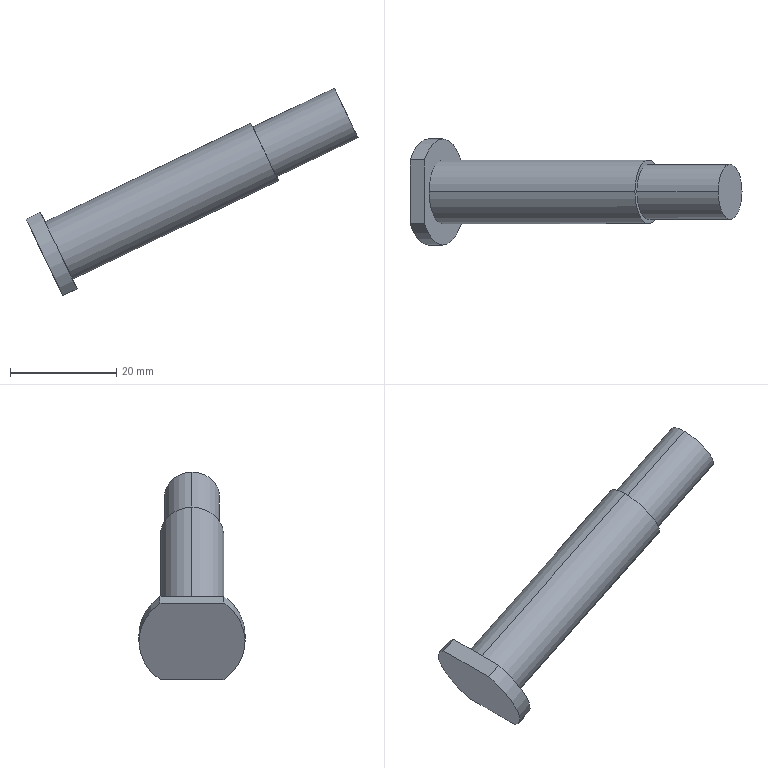Component | SolidWorks | DowelPin1-1-2 | 1 solid | 12 faces | box 62.53 x 20 x 39.12 mm | volume 7145 mm3 | cylinder 6 | plane 6 | commonest cylinder face diameters 10.376 x2 12 x2 20 x2
build123d program:
from build123d import *

# Parameters (mm, degrees)
SKETCH1_R           = 10
BOSS_EXTRUDE1_DEPTH = 3
SKETCH2_R           = 6
BOSS_EXTRUDE2_DEPTH = 43
SKETCH3_R           = 5.188
BOSS_EXTRUDE3_DEPTH = 17
SKETCH4_OUTSIDE_W   = 35.812
SKETCH4_OUTSIDE_H   = 35.812
SKETCH4_OUTSIDE_W_2 = 16
SKETCH4_OUTSIDE_H_2 = 33.428
CUT_EXTRUDE1_DEPTH  = 15


with BuildPart() as part:
    # Sketch1 → Boss-Extrude1 (new body)
    with BuildSketch(Plane.XY):
        Circle(SKETCH1_R)
    extrude(amount=BOSS_EXTRUDE1_DEPTH)

    # Sketch2 → Boss-Extrude2 (add)
    with BuildSketch(Plane.XY.offset(3)):
        Circle(SKETCH2_R)
    extrude(amount=BOSS_EXTRUDE2_DEPTH)

    # Sketch3 → Boss-Extrude3 (add)
    with BuildSketch(Plane.XY.offset(46)):
        Circle(SKETCH3_R)
    extrude(amount=BOSS_EXTRUDE3_DEPTH)

    # Sketch4 outside → Cut-Extrude1 (cut)
    with BuildSketch(Plane(origin=(0, 0, 0), x_dir=(-1, 0, 0), z_dir=(0, 0, -1))):
        Rectangle(SKETCH4_OUTSIDE_W, SKETCH4_OUTSIDE_H)
        Rectangle(SKETCH4_OUTSIDE_W_2, SKETCH4_OUTSIDE_H_2, mode=Mode.SUBTRACT)
    extrude(amount=-CUT_EXTRUDE1_DEPTH, mode=Mode.SUBTRACT)


solid = part.part

# Placed as in the assembly
solid = solid.moved(Location((-107.018, 250, 662.143), (0, 64.419, 179.799)))
STEP:
#1=COLOUR_RGB('',0.7922,0.8196,0.9333);
#2=FILL_AREA_STYLE_COLOUR('',#1);
#3=FILL_AREA_STYLE('',(#2));
#4=SURFACE_STYLE_FILL_AREA(#3);
#5=SURFACE_SIDE_STYLE('',(#4));
#6=SURFACE_STYLE_USAGE(.BOTH.,#5);
#7=PRESENTATION_STYLE_ASSIGNMENT((#6));
#8=CARTESIAN_POINT('',(-1.888,9.842,26.955));
#9=VERTEX_POINT('',#8);
#10=CARTESIAN_POINT('',(-2.064,9.843,27.324));
#11=VERTEX_POINT('',#10);
#12=CARTESIAN_POINT('',(-1.976,9.843,27.14));
#13=DIRECTION('',(0.902,-0.,0.4318));
#14=DIRECTION('',(0.4318,-0.003501,-0.902));
#15=AXIS2_PLACEMENT_3D('',#12,#13,#14);
#16=CIRCLE('',#15,0.2043);
#17=EDGE_CURVE('',#9,#11,#16,.T.);
#18=ORIENTED_EDGE('',*,*,#17,.F.);
#19=CARTESIAN_POINT('',(-2.492,9.842,26.666));
#20=VERTEX_POINT('',#19);
#21=CARTESIAN_POINT('',(-1.888,9.842,26.955));
#22=DIRECTION('',(-0.902,0.,-0.4318));
#23=VECTOR('',#22,39.37);
#24=LINE('',#21,#23);
#25=EDGE_CURVE('',#9,#20,#24,.T.);
#26=ORIENTED_EDGE('',*,*,#25,.T.);
#27=CARTESIAN_POINT('',(-2.668,9.843,27.035));
#28=VERTEX_POINT('',#27);
#29=CARTESIAN_POINT('',(-2.58,9.843,26.851));
#30=DIRECTION('',(0.902,-0.,0.4318));
#31=DIRECTION('',(0.4318,-0.003501,-0.902));
#32=AXIS2_PLACEMENT_3D('',#29,#30,#31);
#33=CIRCLE('',#32,0.2043);
#34=EDGE_CURVE('',#20,#28,#33,.T.);
#35=ORIENTED_EDGE('',*,*,#34,.T.);
#36=CARTESIAN_POINT('',(-2.064,9.843,27.324));
#37=DIRECTION('',(-0.902,0.,-0.4318));
#38=VECTOR('',#37,39.37);
#39=LINE('',#36,#38);
#40=EDGE_CURVE('',#11,#28,#39,.T.);
#41=ORIENTED_EDGE('',*,*,#40,.F.);
#42=EDGE_LOOP('',(#18,#26,#35,#41));
#43=FACE_OUTER_BOUND('',#42,.T.);
#44=CARTESIAN_POINT('',(-1.976,9.843,27.14));
#45=DIRECTION('',(-0.902,0.,-0.4318));
#46=DIRECTION('',(-0.4318,0.003501,0.902));
#47=AXIS2_PLACEMENT_3D('',#44,#45,#46);
#48=CYLINDRICAL_SURFACE('',#47,0.2043);
#49=ADVANCED_FACE('',(#43),#48,.T.);
#50=CARTESIAN_POINT('',(-2.478,9.842,26.638));
#51=VERTEX_POINT('',#50);
#52=CARTESIAN_POINT('',(-2.682,9.843,27.064));
#53=VERTEX_POINT('',#52);
#54=CARTESIAN_POINT('',(-2.58,9.843,26.851));
#55=DIRECTION('',(0.902,-0.,0.4318));
#56=DIRECTION('',(0.4318,-0.003501,-0.902));
#57=AXIS2_PLACEMENT_3D('',#54,#55,#56);
#58=CIRCLE('',#57,0.2362);
#59=EDGE_CURVE('',#51,#53,#58,.T.);
#60=ORIENTED_EDGE('',*,*,#59,.F.);
#61=CARTESIAN_POINT('',(-4.005,9.842,25.907));
#62=VERTEX_POINT('',#61);
#63=CARTESIAN_POINT('',(-2.478,9.842,26.638));
#64=DIRECTION('',(-0.902,0.,-0.4318));
#65=VECTOR('',#64,39.37);
#66=LINE('',#63,#65);
#67=EDGE_CURVE('',#51,#62,#66,.T.);
#68=ORIENTED_EDGE('',*,*,#67,.T.);
#69=CARTESIAN_POINT('',(-4.209,9.843,26.333));
#70=VERTEX_POINT('',#69);
#71=CARTESIAN_POINT('',(-4.107,9.843,26.12));
#72=DIRECTION('',(0.902,-0.,0.4318));
#73=DIRECTION('',(0.4318,-0.003501,-0.902));
#74=AXIS2_PLACEMENT_3D('',#71,#72,#73);
#75=CIRCLE('',#74,0.2362);
#76=EDGE_CURVE('',#62,#70,#75,.T.);
#77=ORIENTED_EDGE('',*,*,#76,.T.);
#78=CARTESIAN_POINT('',(-2.682,9.843,27.064));
#79=DIRECTION('',(-0.902,0.,-0.4318));
#80=VECTOR('',#79,39.37);
#81=LINE('',#78,#80);
#82=EDGE_CURVE('',#53,#70,#81,.T.);
#83=ORIENTED_EDGE('',*,*,#82,.F.);
#84=EDGE_LOOP('',(#60,#68,#77,#83));
#85=FACE_OUTER_BOUND('',#84,.T.);
#86=CARTESIAN_POINT('',(-2.58,9.843,26.851));
#87=DIRECTION('',(-0.902,0.,-0.4318));
#88=DIRECTION('',(-0.4318,0.003501,0.902));
#89=AXIS2_PLACEMENT_3D('',#86,#87,#88);
#90=CYLINDRICAL_SURFACE('',#89,0.2362);
#91=ADVANCED_FACE('',(#85),#90,.T.);
#92=CARTESIAN_POINT('',(-4.242,10.08,26.403));
#93=VERTEX_POINT('',#92);
#94=CARTESIAN_POINT('',(-4.349,10.08,26.352));
#95=VERTEX_POINT('',#94);
#96=CARTESIAN_POINT('',(-4.242,10.08,26.403));
#97=DIRECTION('',(-0.902,0.,-0.4318));
#98=VECTOR('',#97,39.37);
#99=LINE('',#96,#98);
#100=EDGE_CURVE('',#93,#95,#99,.T.);
#101=ORIENTED_EDGE('',*,*,#100,.F.);
#102=CARTESIAN_POINT('',(-3.97,10.078,25.835));
#103=VERTEX_POINT('',#102);
#104=CARTESIAN_POINT('',(-4.107,9.843,26.12));
#105=DIRECTION('',(0.902,-0.,0.4318));
#106=DIRECTION('',(0.4318,-0.003501,-0.902));
#107=AXIS2_PLACEMENT_3D('',#104,#105,#106);
#108=CIRCLE('',#107,0.3937);
#109=EDGE_CURVE('',#103,#93,#108,.T.);
#110=ORIENTED_EDGE('',*,*,#109,.F.);
#111=CARTESIAN_POINT('',(-4.077,10.078,25.784));
#112=VERTEX_POINT('',#111);
#113=CARTESIAN_POINT('',(-3.97,10.078,25.835));
#114=DIRECTION('',(0.902,-0.,0.4318));
#115=VECTOR('',#114,39.37);
#116=LINE('',#113,#115);
#117=EDGE_CURVE('',#112,#103,#116,.T.);
#118=ORIENTED_EDGE('',*,*,#117,.F.);
#119=CARTESIAN_POINT('',(-4.213,9.843,26.069));
#120=DIRECTION('',(0.902,-0.,0.4318));
#121=DIRECTION('',(0.4318,-0.003501,-0.902));
#122=AXIS2_PLACEMENT_3D('',#119,#120,#121);
#123=CIRCLE('',#122,0.3937);
#124=EDGE_CURVE('',#112,#95,#123,.T.);
#125=ORIENTED_EDGE('',*,*,#124,.T.);
#126=EDGE_LOOP('',(#101,#110,#118,#125));
#127=FACE_OUTER_BOUND('',#126,.T.);
#128=CARTESIAN_POINT('',(-4.107,9.843,26.12));
#129=DIRECTION('',(-0.902,0.,-0.4318));
#130=DIRECTION('',(-0.4318,0.003501,0.902));
#131=AXIS2_PLACEMENT_3D('',#128,#129,#130);
#132=CYLINDRICAL_SURFACE('',#131,0.3937);
#133=ADVANCED_FACE('',(#127),#132,.T.);
#134=CARTESIAN_POINT('',(-4.35,9.607,26.353));
#135=VERTEX_POINT('',#134);
#136=CARTESIAN_POINT('',(-4.243,9.607,26.404));
#137=VERTEX_POINT('',#136);
#138=CARTESIAN_POINT('',(-4.243,9.607,26.404));
#139=DIRECTION('',(0.902,-0.,0.4318));
#140=VECTOR('',#139,39.37);
#141=LINE('',#138,#140);
#142=EDGE_CURVE('',#135,#137,#141,.T.);
#143=ORIENTED_EDGE('',*,*,#142,.F.);
#144=CARTESIAN_POINT('',(-4.078,9.605,25.785));
#145=VERTEX_POINT('',#144);
#146=CARTESIAN_POINT('',(-4.213,9.843,26.069));
#147=DIRECTION('',(0.902,-0.,0.4318));
#148=DIRECTION('',(0.4318,-0.003501,-0.902));
#149=AXIS2_PLACEMENT_3D('',#146,#147,#148);
#150=CIRCLE('',#149,0.3937);
#151=EDGE_CURVE('',#135,#145,#150,.T.);
#152=ORIENTED_EDGE('',*,*,#151,.T.);
#153=CARTESIAN_POINT('',(-3.971,9.605,25.836));
#154=VERTEX_POINT('',#153);
#155=CARTESIAN_POINT('',(-3.971,9.605,25.836));
#156=DIRECTION('',(-0.902,0.,-0.4318));
#157=VECTOR('',#156,39.37);
#158=LINE('',#155,#157);
#159=EDGE_CURVE('',#154,#145,#158,.T.);
#160=ORIENTED_EDGE('',*,*,#159,.F.);
#161=CARTESIAN_POINT('',(-4.107,9.843,26.12));
#162=DIRECTION('',(0.902,-0.,0.4318));
#163=DIRECTION('',(0.4318,-0.003501,-0.902));
#164=AXIS2_PLACEMENT_3D('',#161,#162,#163);
#165=CIRCLE('',#164,0.3937);
#166=EDGE_CURVE('',#137,#154,#165,.T.);
#167=ORIENTED_EDGE('',*,*,#166,.F.);
#168=EDGE_LOOP('',(#143,#152,#160,#167));
#169=FACE_OUTER_BOUND('',#168,.T.);
#170=CARTESIAN_POINT('',(-4.107,9.843,26.12));
#171=DIRECTION('',(-0.902,0.,-0.4318));
#172=DIRECTION('',(-0.4318,0.003501,0.902));
#173=AXIS2_PLACEMENT_3D('',#170,#171,#172);
#174=CYLINDRICAL_SURFACE('',#173,0.3937);
#175=ADVANCED_FACE('',(#169),#174,.T.);
#176=CARTESIAN_POINT('',(-4.107,9.843,26.12));
#177=DIRECTION('',(0.902,-0.,0.4318));
#178=DIRECTION('',(0.4318,-0.003501,-0.902));
#179=AXIS2_PLACEMENT_3D('',#176,#177,#178);
#180=CIRCLE('',#179,0.2362);
#181=EDGE_CURVE('',#70,#62,#180,.T.);
#182=ORIENTED_EDGE('',*,*,#181,.F.);
#183=ORIENTED_EDGE('',*,*,#76,.F.);
#184=EDGE_LOOP('',(#182,#183));
#185=FACE_BOUND('',#184,.T.);
#186=ORIENTED_EDGE('',*,*,#109,.T.);
#187=CARTESIAN_POINT('',(-4.243,9.844,26.404));
#188=DIRECTION('',(-0.001512,-1.,0.003158));
#189=VECTOR('',#188,39.37);
#190=LINE('',#187,#189);
#191=EDGE_CURVE('',#93,#137,#190,.T.);
#192=ORIENTED_EDGE('',*,*,#191,.T.);
#193=ORIENTED_EDGE('',*,*,#166,.T.);
#194=CARTESIAN_POINT('',(-3.971,9.841,25.836));
#195=DIRECTION('',(0.001512,1.,-0.003158));
#196=VECTOR('',#195,39.37);
#197=LINE('',#194,#196);
#198=EDGE_CURVE('',#154,#103,#197,.T.);
#199=ORIENTED_EDGE('',*,*,#198,.T.);
#200=EDGE_LOOP('',(#186,#192,#193,#199));
#201=FACE_OUTER_BOUND('',#200,.T.);
#202=CARTESIAN_POINT('',(-4.107,9.843,26.12));
#203=DIRECTION('',(0.902,-0.,0.4318));
#204=DIRECTION('',(0.4318,-0.003501,-0.902));
#205=AXIS2_PLACEMENT_3D('',#202,#203,#204);
#206=PLANE('',#205);
#207=ADVANCED_FACE('',(#185,#201),#206,.T.);
#208=CARTESIAN_POINT('',(-4.349,9.844,26.353));
#209=DIRECTION('',(-0.001512,-1.,0.003158));
#210=VECTOR('',#209,39.37);
#211=LINE('',#208,#210);
#212=EDGE_CURVE('',#95,#135,#211,.T.);
#213=ORIENTED_EDGE('',*,*,#212,.F.);
#214=ORIENTED_EDGE('',*,*,#124,.F.);
#215=CARTESIAN_POINT('',(-4.077,9.841,25.785));
#216=DIRECTION('',(0.001512,1.,-0.003158));
#217=VECTOR('',#216,39.37);
#218=LINE('',#215,#217);
#219=EDGE_CURVE('',#145,#112,#218,.T.);
#220=ORIENTED_EDGE('',*,*,#219,.F.);
#221=ORIENTED_EDGE('',*,*,#151,.F.);
#222=EDGE_LOOP('',(#213,#214,#220,#221));
#223=FACE_OUTER_BOUND('',#222,.T.);
#224=CARTESIAN_POINT('',(-4.213,9.843,26.069));
#225=DIRECTION('',(0.902,-0.,0.4318));
#226=DIRECTION('',(0.4318,-0.003501,-0.902));
#227=AXIS2_PLACEMENT_3D('',#224,#225,#226);
#228=PLANE('',#227);
#229=ADVANCED_FACE('',(#223),#228,.F.);
#230=ORIENTED_EDGE('',*,*,#67,.F.);
#231=CARTESIAN_POINT('',(-2.58,9.843,26.851));
#232=DIRECTION('',(0.902,-0.,0.4318));
#233=DIRECTION('',(0.4318,-0.003501,-0.902));
#234=AXIS2_PLACEMENT_3D('',#231,#232,#233);
#235=CIRCLE('',#234,0.2362);
#236=EDGE_CURVE('',#53,#51,#235,.T.);
#237=ORIENTED_EDGE('',*,*,#236,.F.);
#238=ORIENTED_EDGE('',*,*,#82,.T.);
#239=ORIENTED_EDGE('',*,*,#181,.T.);
#240=EDGE_LOOP('',(#230,#237,#238,#239));
#241=FACE_OUTER_BOUND('',#240,.T.);
#242=CARTESIAN_POINT('',(-2.58,9.843,26.851));
#243=DIRECTION('',(-0.902,0.,-0.4318));
#244=DIRECTION('',(-0.4318,0.003501,0.902));
#245=AXIS2_PLACEMENT_3D('',#242,#243,#244);
#246=CYLINDRICAL_SURFACE('',#245,0.2362);
#247=ADVANCED_FACE('',(#241),#246,.T.);
#248=CARTESIAN_POINT('',(-2.58,9.843,26.851));
#249=DIRECTION('',(0.902,-0.,0.4318));
#250=DIRECTION('',(0.4318,-0.003501,-0.902));
#251=AXIS2_PLACEMENT_3D('',#248,#249,#250);
#252=CIRCLE('',#251,0.2043);
#253=EDGE_CURVE('',#28,#20,#252,.T.);
#254=ORIENTED_EDGE('',*,*,#253,.F.);
#255=ORIENTED_EDGE('',*,*,#34,.F.);
#256=EDGE_LOOP('',(#254,#255));
#257=FACE_BOUND('',#256,.T.);
#258=ORIENTED_EDGE('',*,*,#236,.T.);
#259=ORIENTED_EDGE('',*,*,#59,.T.);
#260=EDGE_LOOP('',(#258,#259));
#261=FACE_OUTER_BOUND('',#260,.T.);
#262=CARTESIAN_POINT('',(-2.58,9.843,26.851));
#263=DIRECTION('',(0.902,-0.,0.4318));
#264=DIRECTION('',(0.4318,-0.003501,-0.902));
#265=AXIS2_PLACEMENT_3D('',#262,#263,#264);
#266=PLANE('',#265);
#267=ADVANCED_FACE('',(#257,#261),#266,.T.);
#268=ORIENTED_EDGE('',*,*,#25,.F.);
#269=CARTESIAN_POINT('',(-1.976,9.843,27.14));
#270=DIRECTION('',(0.902,-0.,0.4318));
#271=DIRECTION('',(0.4318,-0.003501,-0.902));
#272=AXIS2_PLACEMENT_3D('',#269,#270,#271);
#273=CIRCLE('',#272,0.2043);
#274=EDGE_CURVE('',#11,#9,#273,.T.);
#275=ORIENTED_EDGE('',*,*,#274,.F.);
#276=ORIENTED_EDGE('',*,*,#40,.T.);
#277=ORIENTED_EDGE('',*,*,#253,.T.);
#278=EDGE_LOOP('',(#268,#275,#276,#277));
#279=FACE_OUTER_BOUND('',#278,.T.);
#280=CARTESIAN_POINT('',(-1.976,9.843,27.14));
#281=DIRECTION('',(-0.902,0.,-0.4318));
#282=DIRECTION('',(-0.4318,0.003501,0.902));
#283=AXIS2_PLACEMENT_3D('',#280,#281,#282);
#284=CYLINDRICAL_SURFACE('',#283,0.2043);
#285=ADVANCED_FACE('',(#279),#284,.T.);
#286=ORIENTED_EDGE('',*,*,#274,.T.);
#287=ORIENTED_EDGE('',*,*,#17,.T.);
#288=EDGE_LOOP('',(#286,#287));
#289=FACE_OUTER_BOUND('',#288,.T.);
#290=CARTESIAN_POINT('',(-1.976,9.843,27.14));
#291=DIRECTION('',(0.902,-0.,0.4318));
#292=DIRECTION('',(0.4318,-0.003501,-0.902));
#293=AXIS2_PLACEMENT_3D('',#290,#291,#292);
#294=PLANE('',#293);
#295=ADVANCED_FACE('',(#289),#294,.T.);
#296=ORIENTED_EDGE('',*,*,#159,.T.);
#297=ORIENTED_EDGE('',*,*,#219,.T.);
#298=ORIENTED_EDGE('',*,*,#117,.T.);
#299=ORIENTED_EDGE('',*,*,#198,.F.);
#300=EDGE_LOOP('',(#296,#297,#298,#299));
#301=FACE_OUTER_BOUND('',#300,.T.);
#302=CARTESIAN_POINT('',(-3.544,10.499,26.037));
#303=DIRECTION('',(0.4318,-0.003501,-0.902));
#304=DIRECTION('',(0.001512,1.,-0.003158));
#305=AXIS2_PLACEMENT_3D('',#302,#303,#304);
#306=PLANE('',#305);
#307=ADVANCED_FACE('',(#301),#306,.T.);
#308=ORIENTED_EDGE('',*,*,#100,.T.);
#309=ORIENTED_EDGE('',*,*,#212,.T.);
#310=ORIENTED_EDGE('',*,*,#142,.T.);
#311=ORIENTED_EDGE('',*,*,#191,.F.);
#312=EDGE_LOOP('',(#308,#309,#310,#311));
#313=FACE_OUTER_BOUND('',#312,.T.);
#314=CARTESIAN_POINT('',(-3.816,10.502,26.606));
#315=DIRECTION('',(-0.4318,0.003501,0.902));
#316=DIRECTION('',(-0.001512,-1.,0.003158));
#317=AXIS2_PLACEMENT_3D('',#314,#315,#316);
#318=PLANE('',#317);
#319=ADVANCED_FACE('',(#313),#318,.T.);
#320=CLOSED_SHELL('',(#49,#91,#133,#175,#207,#229,#247,#267,#285,#295,#307,#319));
#321=MANIFOLD_SOLID_BREP('',#320);
#322=STYLED_ITEM('',(#7),#321);
#323=PRESENTATION_LAYER_ASSIGNMENT('','',(#322));
#324=CARTESIAN_POINT('',(0.,0.,0.));
#325=DIRECTION('',(0.,0.,1.));
#326=DIRECTION('',(1.,0.,0.));
#327=AXIS2_PLACEMENT_3D('',#324,#325,#326);
#328=(LENGTH_UNIT()NAMED_UNIT(*)SI_UNIT($,.METRE.));
#329=LENGTH_MEASURE_WITH_UNIT(LENGTH_MEASURE(0.0254),#328);
#330=DIMENSIONAL_EXPONENTS(1.,0.,0.,0.,0.,0.,0.);
#331=(CONVERSION_BASED_UNIT('',#329)LENGTH_UNIT()NAMED_UNIT(#330));
#332=UNCERTAINTY_MEASURE_WITH_UNIT(LENGTH_MEASURE(0.00001),#331,'','');
#333=(NAMED_UNIT(*)PLANE_ANGLE_UNIT()SI_UNIT($,.RADIAN.));
#334=(NAMED_UNIT(*)SI_UNIT($,.STERADIAN.)SOLID_ANGLE_UNIT());
#335=(GEOMETRIC_REPRESENTATION_CONTEXT(3)GLOBAL_UNCERTAINTY_ASSIGNED_CONTEXT((#332))GLOBAL_UNIT_ASSIGNED_CONTEXT((#331,#333,#334))REPRESENTATION_CONTEXT('',''));
#336=ADVANCED_BREP_SHAPE_REPRESENTATION('',(#321,#327),#335);
#337=(LENGTH_UNIT()NAMED_UNIT(*)SI_UNIT($,.METRE.));
#338=LENGTH_MEASURE_WITH_UNIT(LENGTH_MEASURE(0.0254),#337);
#339=DIMENSIONAL_EXPONENTS(1.,0.,0.,0.,0.,0.,0.);
#340=(CONVERSION_BASED_UNIT('',#338)LENGTH_UNIT()NAMED_UNIT(#339));
#341=UNCERTAINTY_MEASURE_WITH_UNIT(LENGTH_MEASURE(0.00001),#340,'','');
#342=(NAMED_UNIT(*)PLANE_ANGLE_UNIT()SI_UNIT($,.RADIAN.));
#343=(NAMED_UNIT(*)SI_UNIT($,.STERADIAN.)SOLID_ANGLE_UNIT());
#344=(GEOMETRIC_REPRESENTATION_CONTEXT(3)GLOBAL_UNCERTAINTY_ASSIGNED_CONTEXT((#341))GLOBAL_UNIT_ASSIGNED_CONTEXT((#340,#342,#343))REPRESENTATION_CONTEXT('',''));
#345=MECHANICAL_DESIGN_GEOMETRIC_PRESENTATION_REPRESENTATION('',(#322),#344);